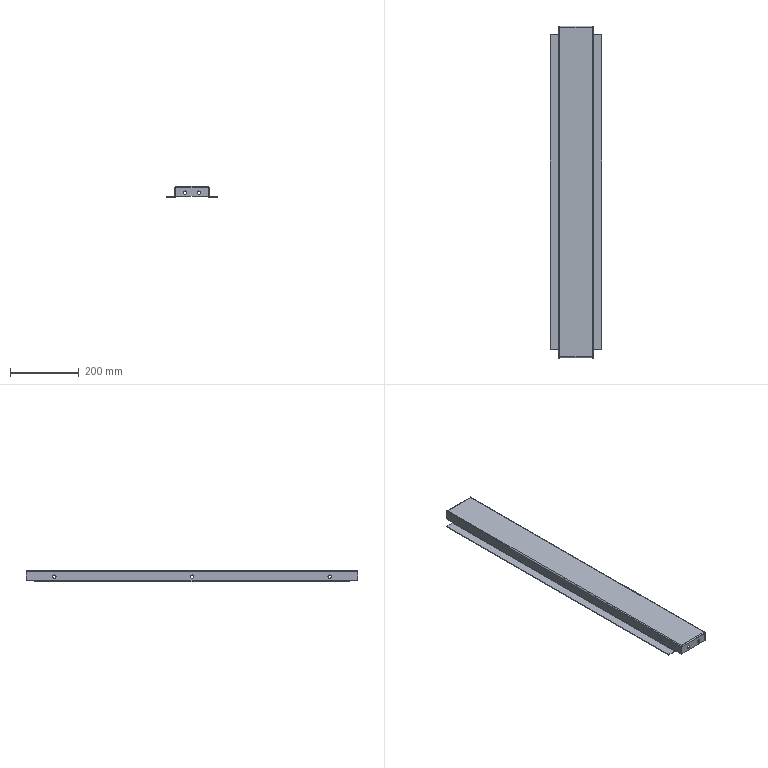Component | SolidWorks | 31FrontMiddleColumn-1 | 1 solid | 82 faces | volume 400910 mm3 | plane 50 | cylinder 32 | commonest cylinder face diameters 10 x20 6 x6 2 x6